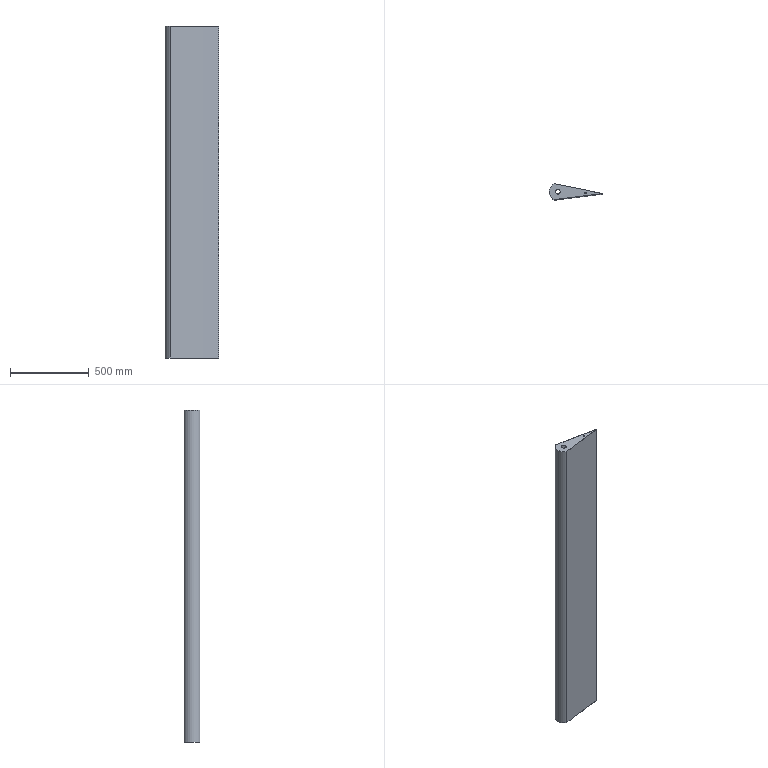Component | NX | AILERON_SKIN | 1 solid | 11 faces | box 341.21 x 101.55 x 2111 mm | volume 799646 mm3 | cylinder 8 | plane 3 | commonest cylinder face diameters 9.808 x1 30 x1 111 x1 43383.705 x1 15525.359 x1 110 x1 43384.705 x1 15524.359 x1
STEP:
#1=CARTESIAN_POINT('',(0.,0.,0.));
#2=DIRECTION('',(0.,0.,1.));
#3=DIRECTION('',(1.,0.,0.));
#4=AXIS2_PLACEMENT_3D('',#1,#2,#3);
#5=CARTESIAN_POINT('',(6874.252,4183.675,-1200.));
#6=VERTEX_POINT('',#5);
#7=CARTESIAN_POINT('',(6869.349,4183.675,-1200.));
#8=DIRECTION('',(0.,0.,-1.));
#9=DIRECTION('',(1.,0.,0.));
#10=AXIS2_PLACEMENT_3D('',#7,#8,#9);
#11=CIRCLE('',#10,4.904);
#12=CARTESIAN_POINT('',(6869.349,4183.675,-3311.));
#13=DIRECTION('',(0.,0.,1.));
#14=DIRECTION('',(1.,0.,0.));
#15=AXIS2_PLACEMENT_3D('',#12,#13,#14);
#16=CYLINDRICAL_SURFACE('',#15,4.904);
#17=CARTESIAN_POINT('',(6.283,2111.));
#18=DIRECTION('',(-1.,0.));
#19=VECTOR('',#18,1.);
#20=LINE('',#17,#19);
#21=(GEOMETRIC_REPRESENTATION_CONTEXT(2)PARAMETRIC_REPRESENTATION_CONTEXT()REPRESENTATION_CONTEXT('',''));
#22=DEFINITIONAL_REPRESENTATION('',(#20),#21);
#23=PCURVE('',#16,#22);
#24=CARTESIAN_POINT('',(8098.679,-6587.303,-1200.));
#25=DIRECTION('',(0.,0.,1.));
#26=DIRECTION('',(1.,0.,0.));
#27=AXIS2_PLACEMENT_3D('',#24,#25,#26);
#28=PLANE('',#27);
#29=CARTESIAN_POINT('',(-1224.427,10770.978));
#30=CARTESIAN_POINT('',(-1224.427,10762.485));
#31=CARTESIAN_POINT('',(-1231.783,10766.731));
#32=CARTESIAN_POINT('',(-1239.138,10770.978));
#33=CARTESIAN_POINT('',(-1231.783,10775.225));
#34=CARTESIAN_POINT('',(-1224.427,10779.472));
#35=CARTESIAN_POINT('',(-1224.427,10770.978));
#36=(BOUNDED_CURVE()B_SPLINE_CURVE(2,(#29,#30,#31,#32,#33,#34,#35),.UNSPECIFIED.,.T.,.F.)B_SPLINE_CURVE_WITH_KNOTS((1,2,2,2,2,1),(-2.094,0.,2.094,4.189,6.283,8.378),.UNSPECIFIED.)CURVE()GEOMETRIC_REPRESENTATION_ITEM()RATIONAL_B_SPLINE_CURVE((1.,0.5,1.,0.5,1.,0.5,1.))REPRESENTATION_ITEM(''));
#37=(GEOMETRIC_REPRESENTATION_CONTEXT(2)PARAMETRIC_REPRESENTATION_CONTEXT()REPRESENTATION_CONTEXT('',''));
#38=DEFINITIONAL_REPRESENTATION('',(#36),#37);
#39=PCURVE('',#28,#38);
#40=SURFACE_CURVE('',#11,(#23,#39),.PCURVE_S1.);
#41=EDGE_CURVE('',#6,#6,#40,.T.);
#42=ORIENTED_EDGE('',*,*,#41,.T.);
#43=CARTESIAN_POINT('',(6874.252,4183.675,-1200.5));
#44=VERTEX_POINT('',#43);
#45=CARTESIAN_POINT('',(6874.252,4183.675,-1200.5));
#46=CARTESIAN_POINT('',(6874.252,4183.675,-1200.));
#47=B_SPLINE_CURVE_WITH_KNOTS('',1,(#45,#46),.UNSPECIFIED.,.F.,.F.,(2,2),(2110.5,2111.),.PIECEWISE_BEZIER_KNOTS.);
#48=CARTESIAN_POINT('',(0.,0.));
#49=DIRECTION('',(0.,1.));
#50=VECTOR('',#49,1.);
#51=LINE('',#48,#50);
#52=(GEOMETRIC_REPRESENTATION_CONTEXT(2)PARAMETRIC_REPRESENTATION_CONTEXT()REPRESENTATION_CONTEXT('',''));
#53=DEFINITIONAL_REPRESENTATION('',(#51),#52);
#54=PCURVE('',#16,#53);
#55=CARTESIAN_POINT('',(6.283,0.));
#56=DIRECTION('',(0.,1.));
#57=VECTOR('',#56,1.);
#58=LINE('',#55,#57);
#59=(GEOMETRIC_REPRESENTATION_CONTEXT(2)PARAMETRIC_REPRESENTATION_CONTEXT()REPRESENTATION_CONTEXT('',''));
#60=DEFINITIONAL_REPRESENTATION('',(#58),#59);
#61=PCURVE('',#16,#60);
#62=SEAM_CURVE('',#47,(#54,#61),.PCURVE_S1.);
#63=EDGE_CURVE('',#44,#6,#62,.T.);
#64=ORIENTED_EDGE('',*,*,#63,.F.);
#65=CARTESIAN_POINT('',(6869.349,4183.675,-1200.5));
#66=DIRECTION('',(0.,0.,-1.));
#67=DIRECTION('',(1.,0.,0.));
#68=AXIS2_PLACEMENT_3D('',#65,#66,#67);
#69=CIRCLE('',#68,4.904);
#70=CARTESIAN_POINT('',(6.283,2110.5));
#71=DIRECTION('',(-1.,0.));
#72=VECTOR('',#71,1.);
#73=LINE('',#70,#72);
#74=(GEOMETRIC_REPRESENTATION_CONTEXT(2)PARAMETRIC_REPRESENTATION_CONTEXT()REPRESENTATION_CONTEXT('',''));
#75=DEFINITIONAL_REPRESENTATION('',(#73),#74);
#76=PCURVE('',#16,#75);
#77=CARTESIAN_POINT('',(8098.679,-6587.303,-1200.5));
#78=DIRECTION('',(0.,0.,1.));
#79=DIRECTION('',(1.,0.,0.));
#80=AXIS2_PLACEMENT_3D('',#77,#78,#79);
#81=PLANE('',#80);
#82=CARTESIAN_POINT('',(-1224.427,10770.978));
#83=CARTESIAN_POINT('',(-1224.427,10762.485));
#84=CARTESIAN_POINT('',(-1231.783,10766.731));
#85=CARTESIAN_POINT('',(-1239.138,10770.978));
#86=CARTESIAN_POINT('',(-1231.783,10775.225));
#87=CARTESIAN_POINT('',(-1224.427,10779.472));
#88=CARTESIAN_POINT('',(-1224.427,10770.978));
#89=(BOUNDED_CURVE()B_SPLINE_CURVE(2,(#82,#83,#84,#85,#86,#87,#88),.UNSPECIFIED.,.T.,.F.)B_SPLINE_CURVE_WITH_KNOTS((1,2,2,2,2,1),(-2.094,0.,2.094,4.189,6.283,8.378),.UNSPECIFIED.)CURVE()GEOMETRIC_REPRESENTATION_ITEM()RATIONAL_B_SPLINE_CURVE((1.,0.5,1.,0.5,1.,0.5,1.))REPRESENTATION_ITEM(''));
#90=(GEOMETRIC_REPRESENTATION_CONTEXT(2)PARAMETRIC_REPRESENTATION_CONTEXT()REPRESENTATION_CONTEXT('',''));
#91=DEFINITIONAL_REPRESENTATION('',(#89),#90);
#92=PCURVE('',#81,#91);
#93=SURFACE_CURVE('',#69,(#76,#92),.PCURVE_S1.);
#94=EDGE_CURVE('',#44,#44,#93,.T.);
#95=ORIENTED_EDGE('',*,*,#94,.F.);
#96=ORIENTED_EDGE('',*,*,#63,.T.);
#97=EDGE_LOOP('',(#42,#64,#95,#96));
#98=FACE_BOUND('',#97,.F.);
#99=ADVANCED_FACE('',(#98),#16,.F.);
#100=CARTESIAN_POINT('',(6709.506,4191.089,-1200.));
#101=VERTEX_POINT('',#100);
#102=CARTESIAN_POINT('',(6694.506,4191.089,-1200.));
#103=DIRECTION('',(0.,0.,-1.));
#104=DIRECTION('',(1.,0.,0.));
#105=AXIS2_PLACEMENT_3D('',#102,#103,#104);
#106=CIRCLE('',#105,15.);
#107=CARTESIAN_POINT('',(6694.506,4191.089,-3311.));
#108=DIRECTION('',(0.,0.,1.));
#109=DIRECTION('',(1.,0.,0.));
#110=AXIS2_PLACEMENT_3D('',#107,#108,#109);
#111=CYLINDRICAL_SURFACE('',#110,15.);
#112=CARTESIAN_POINT('',(6.283,2111.));
#113=DIRECTION('',(-1.,0.));
#114=VECTOR('',#113,1.);
#115=LINE('',#112,#114);
#116=(GEOMETRIC_REPRESENTATION_CONTEXT(2)PARAMETRIC_REPRESENTATION_CONTEXT()REPRESENTATION_CONTEXT('',''));
#117=DEFINITIONAL_REPRESENTATION('',(#115),#116);
#118=PCURVE('',#111,#117);
#119=CARTESIAN_POINT('',(-1389.174,10778.392));
#120=CARTESIAN_POINT('',(-1389.174,10752.411));
#121=CARTESIAN_POINT('',(-1411.674,10765.402));
#122=CARTESIAN_POINT('',(-1434.174,10778.392));
#123=CARTESIAN_POINT('',(-1411.674,10791.382));
#124=CARTESIAN_POINT('',(-1389.174,10804.373));
#125=CARTESIAN_POINT('',(-1389.174,10778.392));
#126=(BOUNDED_CURVE()B_SPLINE_CURVE(2,(#119,#120,#121,#122,#123,#124,#125),.UNSPECIFIED.,.T.,.F.)B_SPLINE_CURVE_WITH_KNOTS((1,2,2,2,2,1),(-2.094,0.,2.094,4.189,6.283,8.378),.UNSPECIFIED.)CURVE()GEOMETRIC_REPRESENTATION_ITEM()RATIONAL_B_SPLINE_CURVE((1.,0.5,1.,0.5,1.,0.5,1.))REPRESENTATION_ITEM(''));
#127=(GEOMETRIC_REPRESENTATION_CONTEXT(2)PARAMETRIC_REPRESENTATION_CONTEXT()REPRESENTATION_CONTEXT('',''));
#128=DEFINITIONAL_REPRESENTATION('',(#126),#127);
#129=PCURVE('',#28,#128);
#130=SURFACE_CURVE('',#106,(#118,#129),.PCURVE_S1.);
#131=EDGE_CURVE('',#101,#101,#130,.T.);
#132=ORIENTED_EDGE('',*,*,#131,.T.);
#133=CARTESIAN_POINT('',(6709.506,4191.089,-1200.5));
#134=VERTEX_POINT('',#133);
#135=CARTESIAN_POINT('',(6709.506,4191.089,-1200.5));
#136=CARTESIAN_POINT('',(6709.506,4191.089,-1200.));
#137=B_SPLINE_CURVE_WITH_KNOTS('',1,(#135,#136),.UNSPECIFIED.,.F.,.F.,(2,2),(2110.5,2111.),.PIECEWISE_BEZIER_KNOTS.);
#138=CARTESIAN_POINT('',(0.,0.));
#139=DIRECTION('',(0.,1.));
#140=VECTOR('',#139,1.);
#141=LINE('',#138,#140);
#142=(GEOMETRIC_REPRESENTATION_CONTEXT(2)PARAMETRIC_REPRESENTATION_CONTEXT()REPRESENTATION_CONTEXT('',''));
#143=DEFINITIONAL_REPRESENTATION('',(#141),#142);
#144=PCURVE('',#111,#143);
#145=CARTESIAN_POINT('',(6.283,0.));
#146=DIRECTION('',(0.,1.));
#147=VECTOR('',#146,1.);
#148=LINE('',#145,#147);
#149=(GEOMETRIC_REPRESENTATION_CONTEXT(2)PARAMETRIC_REPRESENTATION_CONTEXT()REPRESENTATION_CONTEXT('',''));
#150=DEFINITIONAL_REPRESENTATION('',(#148),#149);
#151=PCURVE('',#111,#150);
#152=SEAM_CURVE('',#137,(#144,#151),.PCURVE_S1.);
#153=EDGE_CURVE('',#134,#101,#152,.T.);
#154=ORIENTED_EDGE('',*,*,#153,.F.);
#155=CARTESIAN_POINT('',(6694.506,4191.089,-1200.5));
#156=DIRECTION('',(0.,0.,-1.));
#157=DIRECTION('',(1.,0.,0.));
#158=AXIS2_PLACEMENT_3D('',#155,#156,#157);
#159=CIRCLE('',#158,15.);
#160=CARTESIAN_POINT('',(6.283,2110.5));
#161=DIRECTION('',(-1.,0.));
#162=VECTOR('',#161,1.);
#163=LINE('',#160,#162);
#164=(GEOMETRIC_REPRESENTATION_CONTEXT(2)PARAMETRIC_REPRESENTATION_CONTEXT()REPRESENTATION_CONTEXT('',''));
#165=DEFINITIONAL_REPRESENTATION('',(#163),#164);
#166=PCURVE('',#111,#165);
#167=CARTESIAN_POINT('',(-1389.174,10778.392));
#168=CARTESIAN_POINT('',(-1389.174,10752.411));
#169=CARTESIAN_POINT('',(-1411.674,10765.402));
#170=CARTESIAN_POINT('',(-1434.174,10778.392));
#171=CARTESIAN_POINT('',(-1411.674,10791.382));
#172=CARTESIAN_POINT('',(-1389.174,10804.373));
#173=CARTESIAN_POINT('',(-1389.174,10778.392));
#174=(BOUNDED_CURVE()B_SPLINE_CURVE(2,(#167,#168,#169,#170,#171,#172,#173),.UNSPECIFIED.,.T.,.F.)B_SPLINE_CURVE_WITH_KNOTS((1,2,2,2,2,1),(-2.094,0.,2.094,4.189,6.283,8.378),.UNSPECIFIED.)CURVE()GEOMETRIC_REPRESENTATION_ITEM()RATIONAL_B_SPLINE_CURVE((1.,0.5,1.,0.5,1.,0.5,1.))REPRESENTATION_ITEM(''));
#175=(GEOMETRIC_REPRESENTATION_CONTEXT(2)PARAMETRIC_REPRESENTATION_CONTEXT()REPRESENTATION_CONTEXT('',''));
#176=DEFINITIONAL_REPRESENTATION('',(#174),#175);
#177=PCURVE('',#81,#176);
#178=SURFACE_CURVE('',#159,(#166,#177),.PCURVE_S1.);
#179=EDGE_CURVE('',#134,#134,#178,.T.);
#180=ORIENTED_EDGE('',*,*,#179,.F.);
#181=ORIENTED_EDGE('',*,*,#153,.T.);
#182=EDGE_LOOP('',(#132,#154,#180,#181));
#183=FACE_BOUND('',#182,.F.);
#184=ADVANCED_FACE('',(#183),#111,.F.);
#185=CARTESIAN_POINT('',(6672.701,4242.126,-1200.));
#186=VERTEX_POINT('',#185);
#187=CARTESIAN_POINT('',(6671.501,4140.581,-1200.));
#188=VERTEX_POINT('',#187);
#189=CARTESIAN_POINT('',(6694.506,4191.089,-1200.));
#190=DIRECTION('',(0.,0.,1.));
#191=DIRECTION('',(1.,0.,0.));
#192=AXIS2_PLACEMENT_3D('',#189,#190,#191);
#193=CIRCLE('',#192,55.5);
#194=CARTESIAN_POINT('',(6694.506,4191.089,-3311.));
#195=DIRECTION('',(0.,0.,1.));
#196=DIRECTION('',(1.,0.,0.));
#197=AXIS2_PLACEMENT_3D('',#194,#195,#196);
#198=CYLINDRICAL_SURFACE('',#197,55.5);
#199=CARTESIAN_POINT('',(-0.,2111.));
#200=DIRECTION('',(1.,0.));
#201=VECTOR('',#200,1.);
#202=LINE('',#199,#201);
#203=(GEOMETRIC_REPRESENTATION_CONTEXT(2)PARAMETRIC_REPRESENTATION_CONTEXT()REPRESENTATION_CONTEXT('',''));
#204=DEFINITIONAL_REPRESENTATION('',(#202),#203);
#205=PCURVE('',#198,#204);
#206=CARTESIAN_POINT('',(-1404.174,10778.392));
#207=DIRECTION('',(1.,0.));
#208=AXIS2_PLACEMENT_2D('',#206,#207);
#209=CIRCLE('',#208,55.5);
#210=(GEOMETRIC_REPRESENTATION_CONTEXT(2)PARAMETRIC_REPRESENTATION_CONTEXT()REPRESENTATION_CONTEXT('',''));
#211=DEFINITIONAL_REPRESENTATION('',(#209),#210);
#212=PCURVE('',#28,#211);
#213=SURFACE_CURVE('',#193,(#205,#212),.PCURVE_S1.);
#214=EDGE_CURVE('',#186,#188,#213,.T.);
#215=ORIENTED_EDGE('',*,*,#214,.F.);
#216=CARTESIAN_POINT('',(6672.701,4242.126,-3311.));
#217=VERTEX_POINT('',#216);
#218=CARTESIAN_POINT('',(6672.701,4242.126,-3311.));
#219=DIRECTION('',(0.,0.,1.));
#220=VECTOR('',#219,1.);
#221=LINE('',#218,#220);
#222=CARTESIAN_POINT('',(1.975,0.));
#223=DIRECTION('',(0.,1.));
#224=VECTOR('',#223,1.);
#225=LINE('',#222,#224);
#226=(GEOMETRIC_REPRESENTATION_CONTEXT(2)PARAMETRIC_REPRESENTATION_CONTEXT()REPRESENTATION_CONTEXT('',''));
#227=DEFINITIONAL_REPRESENTATION('',(#225),#226);
#228=PCURVE('',#198,#227);
#229=CARTESIAN_POINT('',(5265.201,-3391.886,-3311.));
#230=DIRECTION('',(0.,0.,1.));
#231=DIRECTION('',(1.,0.,0.));
#232=AXIS2_PLACEMENT_3D('',#229,#230,#231);
#233=CYLINDRICAL_SURFACE('',#232,7762.68);
#234=CARTESIAN_POINT('',(1.388,0.));
#235=DIRECTION('',(0.,1.));
#236=VECTOR('',#235,1.);
#237=LINE('',#234,#236);
#238=(GEOMETRIC_REPRESENTATION_CONTEXT(2)PARAMETRIC_REPRESENTATION_CONTEXT()REPRESENTATION_CONTEXT('',''));
#239=DEFINITIONAL_REPRESENTATION('',(#237),#238);
#240=PCURVE('',#233,#239);
#241=SURFACE_CURVE('',#221,(#228,#240),.PCURVE_S1.);
#242=EDGE_CURVE('',#217,#186,#241,.T.);
#243=ORIENTED_EDGE('',*,*,#242,.F.);
#244=CARTESIAN_POINT('',(6671.501,4140.581,-3311.));
#245=VERTEX_POINT('',#244);
#246=CARTESIAN_POINT('',(6694.506,4191.089,-3311.));
#247=DIRECTION('',(0.,0.,1.));
#248=DIRECTION('',(1.,0.,0.));
#249=AXIS2_PLACEMENT_3D('',#246,#247,#248);
#250=CIRCLE('',#249,55.5);
#251=CARTESIAN_POINT('',(-0.,0.));
#252=DIRECTION('',(1.,0.));
#253=VECTOR('',#252,1.);
#254=LINE('',#251,#253);
#255=(GEOMETRIC_REPRESENTATION_CONTEXT(2)PARAMETRIC_REPRESENTATION_CONTEXT()REPRESENTATION_CONTEXT('',''));
#256=DEFINITIONAL_REPRESENTATION('',(#254),#255);
#257=PCURVE('',#198,#256);
#258=CARTESIAN_POINT('',(8098.679,-6587.303,-3311.));
#259=DIRECTION('',(0.,0.,1.));
#260=DIRECTION('',(1.,0.,0.));
#261=AXIS2_PLACEMENT_3D('',#258,#259,#260);
#262=PLANE('',#261);
#263=CARTESIAN_POINT('',(-1404.174,10778.392));
#264=DIRECTION('',(1.,0.));
#265=AXIS2_PLACEMENT_2D('',#263,#264);
#266=CIRCLE('',#265,55.5);
#267=(GEOMETRIC_REPRESENTATION_CONTEXT(2)PARAMETRIC_REPRESENTATION_CONTEXT()REPRESENTATION_CONTEXT('',''));
#268=DEFINITIONAL_REPRESENTATION('',(#266),#267);
#269=PCURVE('',#262,#268);
#270=SURFACE_CURVE('',#250,(#257,#269),.PCURVE_S1.);
#271=EDGE_CURVE('',#217,#245,#270,.T.);
#272=ORIENTED_EDGE('',*,*,#271,.T.);
#273=CARTESIAN_POINT('',(6671.501,4140.581,-3311.));
#274=DIRECTION('',(0.,0.,1.));
#275=VECTOR('',#274,1.);
#276=LINE('',#273,#275);
#277=CARTESIAN_POINT('',(4.285,0.));
#278=DIRECTION('',(0.,1.));
#279=VECTOR('',#278,1.);
#280=LINE('',#277,#279);
#281=(GEOMETRIC_REPRESENTATION_CONTEXT(2)PARAMETRIC_REPRESENTATION_CONTEXT()REPRESENTATION_CONTEXT('',''));
#282=DEFINITIONAL_REPRESENTATION('',(#280),#281);
#283=PCURVE('',#198,#282);
#284=CARTESIAN_POINT('',(9502.853,-17365.695,-3311.));
#285=DIRECTION('',(0.,0.,1.));
#286=DIRECTION('',(1.,0.,0.));
#287=AXIS2_PLACEMENT_3D('',#284,#285,#286);
#288=CYLINDRICAL_SURFACE('',#287,21691.852);
#289=CARTESIAN_POINT('',(1.702,0.));
#290=DIRECTION('',(0.,1.));
#291=VECTOR('',#290,1.);
#292=LINE('',#289,#291);
#293=(GEOMETRIC_REPRESENTATION_CONTEXT(2)PARAMETRIC_REPRESENTATION_CONTEXT()REPRESENTATION_CONTEXT('',''));
#294=DEFINITIONAL_REPRESENTATION('',(#292),#293);
#295=PCURVE('',#288,#294);
#296=SURFACE_CURVE('',#276,(#283,#295),.PCURVE_S1.);
#297=EDGE_CURVE('',#245,#188,#296,.T.);
#298=ORIENTED_EDGE('',*,*,#297,.T.);
#299=EDGE_LOOP('',(#215,#243,#272,#298));
#300=FACE_BOUND('',#299,.T.);
#301=ADVANCED_FACE('',(#300),#198,.T.);
#302=CARTESIAN_POINT('',(6980.217,4178.974,-3311.));
#303=VERTEX_POINT('',#302);
#304=CARTESIAN_POINT('',(6980.217,4178.974,-1200.));
#305=VERTEX_POINT('',#304);
#306=CARTESIAN_POINT('',(6980.217,4178.974,-3311.));
#307=DIRECTION('',(0.,0.,1.));
#308=VECTOR('',#307,1.);
#309=LINE('',#306,#308);
#310=CARTESIAN_POINT('',(1.687,0.));
#311=DIRECTION('',(0.,1.));
#312=VECTOR('',#311,1.);
#313=LINE('',#310,#312);
#314=(GEOMETRIC_REPRESENTATION_CONTEXT(2)PARAMETRIC_REPRESENTATION_CONTEXT()REPRESENTATION_CONTEXT('',''));
#315=DEFINITIONAL_REPRESENTATION('',(#313),#314);
#316=PCURVE('',#288,#315);
#317=CARTESIAN_POINT('',(1.348,0.));
#318=DIRECTION('',(0.,1.));
#319=VECTOR('',#318,1.);
#320=LINE('',#317,#319);
#321=(GEOMETRIC_REPRESENTATION_CONTEXT(2)PARAMETRIC_REPRESENTATION_CONTEXT()REPRESENTATION_CONTEXT('',''));
#322=DEFINITIONAL_REPRESENTATION('',(#320),#321);
#323=PCURVE('',#233,#322);
#324=SURFACE_CURVE('',#309,(#316,#323),.PCURVE_S1.);
#325=EDGE_CURVE('',#303,#305,#324,.T.);
#326=ORIENTED_EDGE('',*,*,#325,.F.);
#327=CARTESIAN_POINT('',(9502.853,-17365.695,-3311.));
#328=DIRECTION('',(0.,0.,-1.));
#329=DIRECTION('',(1.,0.,0.));
#330=AXIS2_PLACEMENT_3D('',#327,#328,#329);
#331=CIRCLE('',#330,21691.852);
#332=CARTESIAN_POINT('',(6.283,0.));
#333=DIRECTION('',(-1.,0.));
#334=VECTOR('',#333,1.);
#335=LINE('',#332,#334);
#336=(GEOMETRIC_REPRESENTATION_CONTEXT(2)PARAMETRIC_REPRESENTATION_CONTEXT()REPRESENTATION_CONTEXT('',''));
#337=DEFINITIONAL_REPRESENTATION('',(#335),#336);
#338=PCURVE('',#288,#337);
#339=CARTESIAN_POINT('',(23096.026,-10778.392));
#340=CARTESIAN_POINT('',(23096.026,-48349.783));
#341=CARTESIAN_POINT('',(-9441.753,-29564.087));
#342=CARTESIAN_POINT('',(-41979.531,-10778.392));
#343=CARTESIAN_POINT('',(-9441.753,8007.303));
#344=CARTESIAN_POINT('',(23096.026,26792.999));
#345=CARTESIAN_POINT('',(23096.026,-10778.392));
#346=(BOUNDED_CURVE()B_SPLINE_CURVE(2,(#339,#340,#341,#342,#343,#344,#345),.UNSPECIFIED.,.T.,.F.)B_SPLINE_CURVE_WITH_KNOTS((1,2,2,2,2,1),(-2.094,0.,2.094,4.189,6.283,8.378),.UNSPECIFIED.)CURVE()GEOMETRIC_REPRESENTATION_ITEM()RATIONAL_B_SPLINE_CURVE((1.,0.5,1.,0.5,1.,0.5,1.))REPRESENTATION_ITEM(''));
#347=(GEOMETRIC_REPRESENTATION_CONTEXT(2)PARAMETRIC_REPRESENTATION_CONTEXT()REPRESENTATION_CONTEXT('',''));
#348=DEFINITIONAL_REPRESENTATION('',(#346),#347);
#349=PCURVE('',#262,#348);
#350=SURFACE_CURVE('',#331,(#338,#349),.PCURVE_S1.);
#351=EDGE_CURVE('',#245,#303,#350,.T.);
#352=ORIENTED_EDGE('',*,*,#351,.F.);
#353=ORIENTED_EDGE('',*,*,#297,.T.);
#354=CARTESIAN_POINT('',(9502.853,-17365.695,-1200.));
#355=DIRECTION('',(0.,0.,-1.));
#356=DIRECTION('',(1.,0.,0.));
#357=AXIS2_PLACEMENT_3D('',#354,#355,#356);
#358=CIRCLE('',#357,21691.852);
#359=CARTESIAN_POINT('',(6.283,2111.));
#360=DIRECTION('',(-1.,0.));
#361=VECTOR('',#360,1.);
#362=LINE('',#359,#361);
#363=(GEOMETRIC_REPRESENTATION_CONTEXT(2)PARAMETRIC_REPRESENTATION_CONTEXT()REPRESENTATION_CONTEXT('',''));
#364=DEFINITIONAL_REPRESENTATION('',(#362),#363);
#365=PCURVE('',#288,#364);
#366=CARTESIAN_POINT('',(23096.026,-10778.392));
#367=CARTESIAN_POINT('',(23096.026,-48349.783));
#368=CARTESIAN_POINT('',(-9441.753,-29564.087));
#369=CARTESIAN_POINT('',(-41979.531,-10778.392));
#370=CARTESIAN_POINT('',(-9441.753,8007.303));
#371=CARTESIAN_POINT('',(23096.026,26792.999));
#372=CARTESIAN_POINT('',(23096.026,-10778.392));
#373=(BOUNDED_CURVE()B_SPLINE_CURVE(2,(#366,#367,#368,#369,#370,#371,#372),.UNSPECIFIED.,.T.,.F.)B_SPLINE_CURVE_WITH_KNOTS((1,2,2,2,2,1),(-2.094,0.,2.094,4.189,6.283,8.378),.UNSPECIFIED.)CURVE()GEOMETRIC_REPRESENTATION_ITEM()RATIONAL_B_SPLINE_CURVE((1.,0.5,1.,0.5,1.,0.5,1.))REPRESENTATION_ITEM(''));
#374=(GEOMETRIC_REPRESENTATION_CONTEXT(2)PARAMETRIC_REPRESENTATION_CONTEXT()REPRESENTATION_CONTEXT('',''));
#375=DEFINITIONAL_REPRESENTATION('',(#373),#374);
#376=PCURVE('',#28,#375);
#377=SURFACE_CURVE('',#358,(#365,#376),.PCURVE_S1.);
#378=EDGE_CURVE('',#188,#305,#377,.T.);
#379=ORIENTED_EDGE('',*,*,#378,.T.);
#380=EDGE_LOOP('',(#326,#352,#353,#379));
#381=FACE_BOUND('',#380,.F.);
#382=ADVANCED_FACE('',(#381),#288,.F.);
#383=CARTESIAN_POINT('',(5265.201,-3391.886,-1200.));
#384=DIRECTION('',(0.,0.,1.));
#385=DIRECTION('',(-1.,0.,0.));
#386=AXIS2_PLACEMENT_3D('',#383,#384,#385);
#387=CIRCLE('',#386,7762.68);
#388=CARTESIAN_POINT('',(-3.142,2111.));
#389=DIRECTION('',(1.,0.));
#390=VECTOR('',#389,1.);
#391=LINE('',#388,#390);
#392=(GEOMETRIC_REPRESENTATION_CONTEXT(2)PARAMETRIC_REPRESENTATION_CONTEXT()REPRESENTATION_CONTEXT('',''));
#393=DEFINITIONAL_REPRESENTATION('',(#391),#392);
#394=PCURVE('',#233,#393);
#395=CARTESIAN_POINT('',(-2833.478,3195.417));
#396=DIRECTION('',(-1.,0.));
#397=AXIS2_PLACEMENT_2D('',#395,#396);
#398=CIRCLE('',#397,7762.68);
#399=(GEOMETRIC_REPRESENTATION_CONTEXT(2)PARAMETRIC_REPRESENTATION_CONTEXT()REPRESENTATION_CONTEXT('',''));
#400=DEFINITIONAL_REPRESENTATION('',(#398),#399);
#401=PCURVE('',#28,#400);
#402=SURFACE_CURVE('',#387,(#394,#401),.PCURVE_S1.);
#403=EDGE_CURVE('',#305,#186,#402,.T.);
#404=ORIENTED_EDGE('',*,*,#403,.F.);
#405=ORIENTED_EDGE('',*,*,#325,.F.);
#406=CARTESIAN_POINT('',(5265.201,-3391.886,-3311.));
#407=DIRECTION('',(0.,0.,1.));
#408=DIRECTION('',(-1.,0.,0.));
#409=AXIS2_PLACEMENT_3D('',#406,#407,#408);
#410=CIRCLE('',#409,7762.68);
#411=CARTESIAN_POINT('',(-3.142,0.));
#412=DIRECTION('',(1.,0.));
#413=VECTOR('',#412,1.);
#414=LINE('',#411,#413);
#415=(GEOMETRIC_REPRESENTATION_CONTEXT(2)PARAMETRIC_REPRESENTATION_CONTEXT()REPRESENTATION_CONTEXT('',''));
#416=DEFINITIONAL_REPRESENTATION('',(#414),#415);
#417=PCURVE('',#233,#416);
#418=CARTESIAN_POINT('',(-2833.478,3195.417));
#419=DIRECTION('',(-1.,0.));
#420=AXIS2_PLACEMENT_2D('',#418,#419);
#421=CIRCLE('',#420,7762.68);
#422=(GEOMETRIC_REPRESENTATION_CONTEXT(2)PARAMETRIC_REPRESENTATION_CONTEXT()REPRESENTATION_CONTEXT('',''));
#423=DEFINITIONAL_REPRESENTATION('',(#421),#422);
#424=PCURVE('',#262,#423);
#425=SURFACE_CURVE('',#410,(#417,#424),.PCURVE_S1.);
#426=EDGE_CURVE('',#303,#217,#425,.T.);
#427=ORIENTED_EDGE('',*,*,#426,.T.);
#428=ORIENTED_EDGE('',*,*,#242,.T.);
#429=EDGE_LOOP('',(#404,#405,#427,#428));
#430=FACE_BOUND('',#429,.T.);
#431=ADVANCED_FACE('',(#430),#233,.T.);
#432=CARTESIAN_POINT('',(6977.259,4179.131,-3311.));
#433=VERTEX_POINT('',#432);
#434=CARTESIAN_POINT('',(6672.759,4241.607,-3311.));
#435=VERTEX_POINT('',#434);
#436=CARTESIAN_POINT('',(5265.201,-3391.886,-3311.));
#437=DIRECTION('',(0.,0.,1.));
#438=DIRECTION('',(1.,0.,0.));
#439=AXIS2_PLACEMENT_3D('',#436,#437,#438);
#440=CIRCLE('',#439,7762.18);
#441=CARTESIAN_POINT('',(-2833.478,3195.417));
#442=DIRECTION('',(1.,0.));
#443=AXIS2_PLACEMENT_2D('',#441,#442);
#444=CIRCLE('',#443,7762.18);
#445=(GEOMETRIC_REPRESENTATION_CONTEXT(2)PARAMETRIC_REPRESENTATION_CONTEXT()REPRESENTATION_CONTEXT('',''));
#446=DEFINITIONAL_REPRESENTATION('',(#444),#445);
#447=PCURVE('',#262,#446);
#448=CARTESIAN_POINT('',(5265.201,-3391.886,-3311.));
#449=DIRECTION('',(0.,0.,1.));
#450=DIRECTION('',(1.,0.,0.));
#451=AXIS2_PLACEMENT_3D('',#448,#449,#450);
#452=CYLINDRICAL_SURFACE('',#451,7762.18);
#453=CARTESIAN_POINT('',(0.,0.));
#454=DIRECTION('',(1.,0.));
#455=VECTOR('',#454,1.);
#456=LINE('',#453,#455);
#457=(GEOMETRIC_REPRESENTATION_CONTEXT(2)PARAMETRIC_REPRESENTATION_CONTEXT()REPRESENTATION_CONTEXT('',''));
#458=DEFINITIONAL_REPRESENTATION('',(#456),#457);
#459=PCURVE('',#452,#458);
#460=SURFACE_CURVE('',#440,(#447,#459),.PCURVE_S1.);
#461=EDGE_CURVE('',#433,#435,#460,.T.);
#462=ORIENTED_EDGE('',*,*,#461,.T.);
#463=CARTESIAN_POINT('',(6671.578,4141.096,-3311.));
#464=VERTEX_POINT('',#463);
#465=CARTESIAN_POINT('',(6694.506,4191.089,-3311.));
#466=DIRECTION('',(0.,0.,1.));
#467=DIRECTION('',(1.,0.,0.));
#468=AXIS2_PLACEMENT_3D('',#465,#466,#467);
#469=CIRCLE('',#468,55.);
#470=CARTESIAN_POINT('',(-1404.174,10778.392));
#471=DIRECTION('',(1.,0.));
#472=AXIS2_PLACEMENT_2D('',#470,#471);
#473=CIRCLE('',#472,55.);
#474=(GEOMETRIC_REPRESENTATION_CONTEXT(2)PARAMETRIC_REPRESENTATION_CONTEXT()REPRESENTATION_CONTEXT('',''));
#475=DEFINITIONAL_REPRESENTATION('',(#473),#474);
#476=PCURVE('',#262,#475);
#477=CARTESIAN_POINT('',(6694.506,4191.089,-3311.));
#478=DIRECTION('',(0.,0.,1.));
#479=DIRECTION('',(1.,0.,0.));
#480=AXIS2_PLACEMENT_3D('',#477,#478,#479);
#481=CYLINDRICAL_SURFACE('',#480,55.);
#482=CARTESIAN_POINT('',(-0.,0.));
#483=DIRECTION('',(1.,0.));
#484=VECTOR('',#483,1.);
#485=LINE('',#482,#484);
#486=(GEOMETRIC_REPRESENTATION_CONTEXT(2)PARAMETRIC_REPRESENTATION_CONTEXT()REPRESENTATION_CONTEXT('',''));
#487=DEFINITIONAL_REPRESENTATION('',(#485),#486);
#488=PCURVE('',#481,#487);
#489=SURFACE_CURVE('',#469,(#476,#488),.PCURVE_S1.);
#490=EDGE_CURVE('',#435,#464,#489,.T.);
#491=ORIENTED_EDGE('',*,*,#490,.T.);
#492=CARTESIAN_POINT('',(9502.853,-17365.695,-3311.));
#493=DIRECTION('',(0.,0.,-1.));
#494=DIRECTION('',(1.,0.,0.));
#495=AXIS2_PLACEMENT_3D('',#492,#493,#494);
#496=CIRCLE('',#495,21692.352);
#497=CARTESIAN_POINT('',(23096.526,-10778.392));
#498=CARTESIAN_POINT('',(23096.526,-48350.649));
#499=CARTESIAN_POINT('',(-9442.003,-29564.52));
#500=CARTESIAN_POINT('',(-41980.531,-10778.392));
#501=CARTESIAN_POINT('',(-9442.003,8007.736));
#502=CARTESIAN_POINT('',(23096.526,26793.865));
#503=CARTESIAN_POINT('',(23096.526,-10778.392));
#504=(BOUNDED_CURVE()B_SPLINE_CURVE(2,(#497,#498,#499,#500,#501,#502,#503),.UNSPECIFIED.,.T.,.F.)B_SPLINE_CURVE_WITH_KNOTS((1,2,2,2,2,1),(-2.094,0.,2.094,4.189,6.283,8.378),.UNSPECIFIED.)CURVE()GEOMETRIC_REPRESENTATION_ITEM()RATIONAL_B_SPLINE_CURVE((1.,0.5,1.,0.5,1.,0.5,1.))REPRESENTATION_ITEM(''));
#505=(GEOMETRIC_REPRESENTATION_CONTEXT(2)PARAMETRIC_REPRESENTATION_CONTEXT()REPRESENTATION_CONTEXT('',''));
#506=DEFINITIONAL_REPRESENTATION('',(#504),#505);
#507=PCURVE('',#262,#506);
#508=CARTESIAN_POINT('',(9502.853,-17365.695,-3311.));
#509=DIRECTION('',(0.,0.,1.));
#510=DIRECTION('',(1.,0.,0.));
#511=AXIS2_PLACEMENT_3D('',#508,#509,#510);
#512=CYLINDRICAL_SURFACE('',#511,21692.352);
#513=CARTESIAN_POINT('',(6.283,0.));
#514=DIRECTION('',(-1.,0.));
#515=VECTOR('',#514,1.);
#516=LINE('',#513,#515);
#517=(GEOMETRIC_REPRESENTATION_CONTEXT(2)PARAMETRIC_REPRESENTATION_CONTEXT()REPRESENTATION_CONTEXT('',''));
#518=DEFINITIONAL_REPRESENTATION('',(#516),#517);
#519=PCURVE('',#512,#518);
#520=SURFACE_CURVE('',#496,(#507,#519),.PCURVE_S1.);
#521=EDGE_CURVE('',#464,#433,#520,.T.);
#522=ORIENTED_EDGE('',*,*,#521,.T.);
#523=EDGE_LOOP('',(#462,#491,#522));
#524=FACE_BOUND('',#523,.T.);
#525=ORIENTED_EDGE('',*,*,#271,.F.);
#526=ORIENTED_EDGE('',*,*,#426,.F.);
#527=ORIENTED_EDGE('',*,*,#351,.F.);
#528=EDGE_LOOP('',(#525,#526,#527));
#529=FACE_BOUND('',#528,.T.);
#530=ADVANCED_FACE('',(#524,#529),#262,.F.);
#531=ORIENTED_EDGE('',*,*,#214,.T.);
#532=ORIENTED_EDGE('',*,*,#378,.T.);
#533=ORIENTED_EDGE('',*,*,#403,.T.);
#534=EDGE_LOOP('',(#531,#532,#533));
#535=FACE_BOUND('',#534,.T.);
#536=ORIENTED_EDGE('',*,*,#41,.T.);
#537=EDGE_LOOP('',(#536));
#538=FACE_BOUND('',#537,.T.);
#539=ORIENTED_EDGE('',*,*,#131,.T.);
#540=EDGE_LOOP('',(#539));
#541=FACE_BOUND('',#540,.T.);
#542=ADVANCED_FACE('',(#535,#538,#541),#28,.T.);
#543=CARTESIAN_POINT('',(6672.759,4241.607,-1200.5));
#544=VERTEX_POINT('',#543);
#545=CARTESIAN_POINT('',(6672.759,4241.607,-3311.));
#546=DIRECTION('',(0.,0.,1.));
#547=VECTOR('',#546,1.);
#548=LINE('',#545,#547);
#549=CARTESIAN_POINT('',(1.977,0.));
#550=DIRECTION('',(0.,1.));
#551=VECTOR('',#550,1.);
#552=LINE('',#549,#551);
#553=(GEOMETRIC_REPRESENTATION_CONTEXT(2)PARAMETRIC_REPRESENTATION_CONTEXT()REPRESENTATION_CONTEXT('',''));
#554=DEFINITIONAL_REPRESENTATION('',(#552),#553);
#555=PCURVE('',#481,#554);
#556=CARTESIAN_POINT('',(1.388,0.));
#557=DIRECTION('',(0.,1.));
#558=VECTOR('',#557,1.);
#559=LINE('',#556,#558);
#560=(GEOMETRIC_REPRESENTATION_CONTEXT(2)PARAMETRIC_REPRESENTATION_CONTEXT()REPRESENTATION_CONTEXT('',''));
#561=DEFINITIONAL_REPRESENTATION('',(#559),#560);
#562=PCURVE('',#452,#561);
#563=SURFACE_CURVE('',#548,(#555,#562),.PCURVE_S1.);
#564=EDGE_CURVE('',#435,#544,#563,.T.);
#565=ORIENTED_EDGE('',*,*,#564,.F.);
#566=ORIENTED_EDGE('',*,*,#490,.T.);
#567=CARTESIAN_POINT('',(6671.578,4141.096,-1200.5));
#568=VERTEX_POINT('',#567);
#569=CARTESIAN_POINT('',(6671.578,4141.096,-3311.));
#570=DIRECTION('',(0.,0.,1.));
#571=VECTOR('',#570,1.);
#572=LINE('',#569,#571);
#573=CARTESIAN_POINT('',(4.282,0.));
#574=DIRECTION('',(0.,1.));
#575=VECTOR('',#574,1.);
#576=LINE('',#573,#575);
#577=(GEOMETRIC_REPRESENTATION_CONTEXT(2)PARAMETRIC_REPRESENTATION_CONTEXT()REPRESENTATION_CONTEXT('',''));
#578=DEFINITIONAL_REPRESENTATION('',(#576),#577);
#579=PCURVE('',#481,#578);
#580=CARTESIAN_POINT('',(1.702,0.));
#581=DIRECTION('',(0.,1.));
#582=VECTOR('',#581,1.);
#583=LINE('',#580,#582);
#584=(GEOMETRIC_REPRESENTATION_CONTEXT(2)PARAMETRIC_REPRESENTATION_CONTEXT()REPRESENTATION_CONTEXT('',''));
#585=DEFINITIONAL_REPRESENTATION('',(#583),#584);
#586=PCURVE('',#512,#585);
#587=SURFACE_CURVE('',#572,(#579,#586),.PCURVE_S1.);
#588=EDGE_CURVE('',#464,#568,#587,.T.);
#589=ORIENTED_EDGE('',*,*,#588,.T.);
#590=CARTESIAN_POINT('',(6694.506,4191.089,-1200.5));
#591=DIRECTION('',(0.,0.,1.));
#592=DIRECTION('',(1.,0.,0.));
#593=AXIS2_PLACEMENT_3D('',#590,#591,#592);
#594=CIRCLE('',#593,55.);
#595=CARTESIAN_POINT('',(-0.,2110.5));
#596=DIRECTION('',(1.,0.));
#597=VECTOR('',#596,1.);
#598=LINE('',#595,#597);
#599=(GEOMETRIC_REPRESENTATION_CONTEXT(2)PARAMETRIC_REPRESENTATION_CONTEXT()REPRESENTATION_CONTEXT('',''));
#600=DEFINITIONAL_REPRESENTATION('',(#598),#599);
#601=PCURVE('',#481,#600);
#602=CARTESIAN_POINT('',(-1404.174,10778.392));
#603=DIRECTION('',(1.,0.));
#604=AXIS2_PLACEMENT_2D('',#602,#603);
#605=CIRCLE('',#604,55.);
#606=(GEOMETRIC_REPRESENTATION_CONTEXT(2)PARAMETRIC_REPRESENTATION_CONTEXT()REPRESENTATION_CONTEXT('',''));
#607=DEFINITIONAL_REPRESENTATION('',(#605),#606);
#608=PCURVE('',#81,#607);
#609=SURFACE_CURVE('',#594,(#601,#608),.PCURVE_S1.);
#610=EDGE_CURVE('',#544,#568,#609,.T.);
#611=ORIENTED_EDGE('',*,*,#610,.F.);
#612=EDGE_LOOP('',(#565,#566,#589,#611));
#613=FACE_BOUND('',#612,.F.);
#614=ADVANCED_FACE('',(#613),#481,.F.);
#615=CARTESIAN_POINT('',(6977.259,4179.131,-1200.5));
#616=VERTEX_POINT('',#615);
#617=CARTESIAN_POINT('',(9502.853,-17365.695,-1200.5));
#618=DIRECTION('',(0.,0.,-1.));
#619=DIRECTION('',(1.,0.,0.));
#620=AXIS2_PLACEMENT_3D('',#617,#618,#619);
#621=CIRCLE('',#620,21692.352);
#622=CARTESIAN_POINT('',(6.283,2110.5));
#623=DIRECTION('',(-1.,0.));
#624=VECTOR('',#623,1.);
#625=LINE('',#622,#624);
#626=(GEOMETRIC_REPRESENTATION_CONTEXT(2)PARAMETRIC_REPRESENTATION_CONTEXT()REPRESENTATION_CONTEXT('',''));
#627=DEFINITIONAL_REPRESENTATION('',(#625),#626);
#628=PCURVE('',#512,#627);
#629=CARTESIAN_POINT('',(23096.526,-10778.392));
#630=CARTESIAN_POINT('',(23096.526,-48350.649));
#631=CARTESIAN_POINT('',(-9442.003,-29564.52));
#632=CARTESIAN_POINT('',(-41980.531,-10778.392));
#633=CARTESIAN_POINT('',(-9442.003,8007.736));
#634=CARTESIAN_POINT('',(23096.526,26793.865));
#635=CARTESIAN_POINT('',(23096.526,-10778.392));
#636=(BOUNDED_CURVE()B_SPLINE_CURVE(2,(#629,#630,#631,#632,#633,#634,#635),.UNSPECIFIED.,.T.,.F.)B_SPLINE_CURVE_WITH_KNOTS((1,2,2,2,2,1),(-2.094,0.,2.094,4.189,6.283,8.378),.UNSPECIFIED.)CURVE()GEOMETRIC_REPRESENTATION_ITEM()RATIONAL_B_SPLINE_CURVE((1.,0.5,1.,0.5,1.,0.5,1.))REPRESENTATION_ITEM(''));
#637=(GEOMETRIC_REPRESENTATION_CONTEXT(2)PARAMETRIC_REPRESENTATION_CONTEXT()REPRESENTATION_CONTEXT('',''));
#638=DEFINITIONAL_REPRESENTATION('',(#636),#637);
#639=PCURVE('',#81,#638);
#640=SURFACE_CURVE('',#621,(#628,#639),.PCURVE_S1.);
#641=EDGE_CURVE('',#568,#616,#640,.T.);
#642=ORIENTED_EDGE('',*,*,#641,.T.);
#643=CARTESIAN_POINT('',(6977.259,4179.131,-3311.));
#644=DIRECTION('',(0.,0.,1.));
#645=VECTOR('',#644,1.);
#646=LINE('',#643,#645);
#647=CARTESIAN_POINT('',(1.687,0.));
#648=DIRECTION('',(0.,1.));
#649=VECTOR('',#648,1.);
#650=LINE('',#647,#649);
#651=(GEOMETRIC_REPRESENTATION_CONTEXT(2)PARAMETRIC_REPRESENTATION_CONTEXT()REPRESENTATION_CONTEXT('',''));
#652=DEFINITIONAL_REPRESENTATION('',(#650),#651);
#653=PCURVE('',#512,#652);
#654=CARTESIAN_POINT('',(1.348,0.));
#655=DIRECTION('',(0.,1.));
#656=VECTOR('',#655,1.);
#657=LINE('',#654,#656);
#658=(GEOMETRIC_REPRESENTATION_CONTEXT(2)PARAMETRIC_REPRESENTATION_CONTEXT()REPRESENTATION_CONTEXT('',''));
#659=DEFINITIONAL_REPRESENTATION('',(#657),#658);
#660=PCURVE('',#452,#659);
#661=SURFACE_CURVE('',#646,(#653,#660),.PCURVE_S1.);
#662=EDGE_CURVE('',#433,#616,#661,.T.);
#663=ORIENTED_EDGE('',*,*,#662,.F.);
#664=ORIENTED_EDGE('',*,*,#521,.F.);
#665=ORIENTED_EDGE('',*,*,#588,.T.);
#666=EDGE_LOOP('',(#642,#663,#664,#665));
#667=FACE_BOUND('',#666,.T.);
#668=ADVANCED_FACE('',(#667),#512,.T.);
#669=ORIENTED_EDGE('',*,*,#662,.F.);
#670=ORIENTED_EDGE('',*,*,#461,.T.);
#671=ORIENTED_EDGE('',*,*,#564,.T.);
#672=CARTESIAN_POINT('',(5265.201,-3391.886,-1200.5));
#673=DIRECTION('',(0.,0.,1.));
#674=DIRECTION('',(1.,0.,0.));
#675=AXIS2_PLACEMENT_3D('',#672,#673,#674);
#676=CIRCLE('',#675,7762.18);
#677=CARTESIAN_POINT('',(0.,2110.5));
#678=DIRECTION('',(1.,0.));
#679=VECTOR('',#678,1.);
#680=LINE('',#677,#679);
#681=(GEOMETRIC_REPRESENTATION_CONTEXT(2)PARAMETRIC_REPRESENTATION_CONTEXT()REPRESENTATION_CONTEXT('',''));
#682=DEFINITIONAL_REPRESENTATION('',(#680),#681);
#683=PCURVE('',#452,#682);
#684=CARTESIAN_POINT('',(-2833.478,3195.417));
#685=DIRECTION('',(1.,0.));
#686=AXIS2_PLACEMENT_2D('',#684,#685);
#687=CIRCLE('',#686,7762.18);
#688=(GEOMETRIC_REPRESENTATION_CONTEXT(2)PARAMETRIC_REPRESENTATION_CONTEXT()REPRESENTATION_CONTEXT('',''));
#689=DEFINITIONAL_REPRESENTATION('',(#687),#688);
#690=PCURVE('',#81,#689);
#691=SURFACE_CURVE('',#676,(#683,#690),.PCURVE_S1.);
#692=EDGE_CURVE('',#616,#544,#691,.T.);
#693=ORIENTED_EDGE('',*,*,#692,.F.);
#694=EDGE_LOOP('',(#669,#670,#671,#693));
#695=FACE_BOUND('',#694,.F.);
#696=ADVANCED_FACE('',(#695),#452,.F.);
#697=ORIENTED_EDGE('',*,*,#610,.F.);
#698=ORIENTED_EDGE('',*,*,#692,.F.);
#699=ORIENTED_EDGE('',*,*,#641,.F.);
#700=EDGE_LOOP('',(#697,#698,#699));
#701=FACE_BOUND('',#700,.T.);
#702=ORIENTED_EDGE('',*,*,#94,.F.);
#703=EDGE_LOOP('',(#702));
#704=FACE_BOUND('',#703,.T.);
#705=ORIENTED_EDGE('',*,*,#179,.F.);
#706=EDGE_LOOP('',(#705));
#707=FACE_BOUND('',#706,.T.);
#708=ADVANCED_FACE('',(#701,#704,#707),#81,.F.);
#709=CLOSED_SHELL('',(#99,#184,#301,#382,#431,#530,#542,#614,#668,#696,#708));
#710=MANIFOLD_SOLID_BREP('',#709);
#711=(LENGTH_UNIT()NAMED_UNIT(*)SI_UNIT(.MILLI.,.METRE.));
#712=UNCERTAINTY_MEASURE_WITH_UNIT(LENGTH_MEASURE(0.000002),#711,'','');
#713=(NAMED_UNIT(*)PLANE_ANGLE_UNIT()SI_UNIT($,.RADIAN.));
#714=(NAMED_UNIT(*)SI_UNIT($,.STERADIAN.)SOLID_ANGLE_UNIT());
#715=(GEOMETRIC_REPRESENTATION_CONTEXT(3)GLOBAL_UNCERTAINTY_ASSIGNED_CONTEXT((#712))GLOBAL_UNIT_ASSIGNED_CONTEXT((#711,#713,#714))REPRESENTATION_CONTEXT('',''));
#716=ADVANCED_BREP_SHAPE_REPRESENTATION('',(#4,#710),#715);